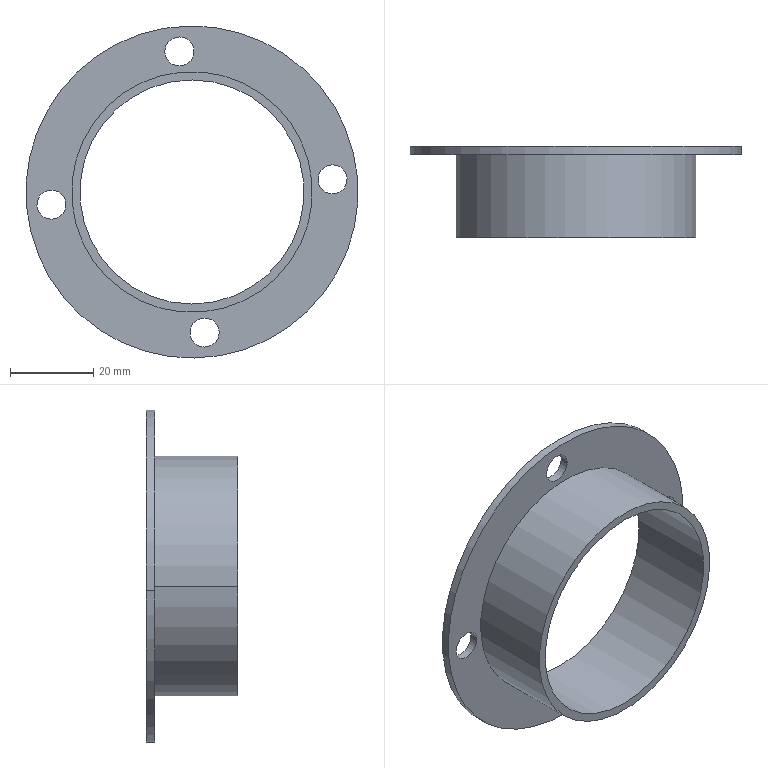Component | SolidWorks | ControllerRotatingShaft-1 | 1 solid | 17 faces | box 80 x 22 x 80 mm | volume 12202 mm3 | cylinder 14 | plane 3 | commonest cylinder face diameters 7 x8 80 x2 54 x2 58 x2
STEP:
#1=COLOUR_RGB('',0.7922,0.8196,0.9333);
#2=FILL_AREA_STYLE_COLOUR('',#1);
#3=FILL_AREA_STYLE('',(#2));
#4=SURFACE_STYLE_FILL_AREA(#3);
#5=SURFACE_SIDE_STYLE('',(#4));
#6=SURFACE_STYLE_USAGE(.BOTH.,#5);
#7=PRESENTATION_STYLE_ASSIGNMENT((#6));
#8=CARTESIAN_POINT('',(13.418,-5.647,18.276));
#9=VERTEX_POINT('',#8);
#10=CARTESIAN_POINT('',(13.693,-5.647,18.3));
#11=VERTEX_POINT('',#10);
#12=CARTESIAN_POINT('',(13.556,-5.647,18.288));
#13=DIRECTION('',(0.,1.,0.));
#14=DIRECTION('',(0.996,0.,0.08937));
#15=AXIS2_PLACEMENT_3D('',#12,#13,#14);
#16=CIRCLE('',#15,0.1378);
#17=EDGE_CURVE('',#9,#11,#16,.T.);
#18=ORIENTED_EDGE('',*,*,#17,.F.);
#19=CARTESIAN_POINT('',(13.418,-5.568,18.276));
#20=VERTEX_POINT('',#19);
#21=CARTESIAN_POINT('',(13.418,-5.962,18.276));
#22=DIRECTION('',(0.,1.,0.));
#23=VECTOR('',#22,39.37);
#24=LINE('',#21,#23);
#25=EDGE_CURVE('',#9,#20,#24,.T.);
#26=ORIENTED_EDGE('',*,*,#25,.T.);
#27=CARTESIAN_POINT('',(13.693,-5.568,18.3));
#28=VERTEX_POINT('',#27);
#29=CARTESIAN_POINT('',(13.556,-5.568,18.288));
#30=DIRECTION('',(0.,1.,0.));
#31=DIRECTION('',(-0.08937,0.,0.996));
#32=AXIS2_PLACEMENT_3D('',#29,#30,#31);
#33=CIRCLE('',#32,0.1378);
#34=EDGE_CURVE('',#20,#28,#33,.T.);
#35=ORIENTED_EDGE('',*,*,#34,.T.);
#36=CARTESIAN_POINT('',(13.693,-5.962,18.3));
#37=DIRECTION('',(0.,1.,0.));
#38=VECTOR('',#37,39.37);
#39=LINE('',#36,#38);
#40=EDGE_CURVE('',#11,#28,#39,.T.);
#41=ORIENTED_EDGE('',*,*,#40,.F.);
#42=EDGE_LOOP('',(#18,#26,#35,#41));
#43=FACE_OUTER_BOUND('',#42,.T.);
#44=CARTESIAN_POINT('',(13.556,-5.962,18.288));
#45=DIRECTION('',(0.,1.,0.));
#46=DIRECTION('',(0.996,0.,0.08937));
#47=AXIS2_PLACEMENT_3D('',#44,#45,#46);
#48=CYLINDRICAL_SURFACE('',#47,0.1378);
#49=ADVANCED_FACE('',(#43),#48,.F.);
#50=CARTESIAN_POINT('',(11.966,-5.647,19.489));
#51=VERTEX_POINT('',#50);
#52=CARTESIAN_POINT('',(12.24,-5.647,19.514));
#53=VERTEX_POINT('',#52);
#54=CARTESIAN_POINT('',(12.103,-5.647,19.502));
#55=DIRECTION('',(0.,1.,0.));
#56=DIRECTION('',(0.996,0.,0.08937));
#57=AXIS2_PLACEMENT_3D('',#54,#55,#56);
#58=CIRCLE('',#57,0.1378);
#59=EDGE_CURVE('',#51,#53,#58,.T.);
#60=ORIENTED_EDGE('',*,*,#59,.F.);
#61=CARTESIAN_POINT('',(11.966,-5.568,19.489));
#62=VERTEX_POINT('',#61);
#63=CARTESIAN_POINT('',(11.966,-5.962,19.489));
#64=DIRECTION('',(0.,1.,0.));
#65=VECTOR('',#64,39.37);
#66=LINE('',#63,#65);
#67=EDGE_CURVE('',#51,#62,#66,.T.);
#68=ORIENTED_EDGE('',*,*,#67,.T.);
#69=CARTESIAN_POINT('',(12.24,-5.568,19.514));
#70=VERTEX_POINT('',#69);
#71=CARTESIAN_POINT('',(12.103,-5.568,19.502));
#72=DIRECTION('',(0.,1.,0.));
#73=DIRECTION('',(-0.996,0.,-0.08937));
#74=AXIS2_PLACEMENT_3D('',#71,#72,#73);
#75=CIRCLE('',#74,0.1378);
#76=EDGE_CURVE('',#62,#70,#75,.T.);
#77=ORIENTED_EDGE('',*,*,#76,.T.);
#78=CARTESIAN_POINT('',(12.24,-5.962,19.514));
#79=DIRECTION('',(0.,1.,0.));
#80=VECTOR('',#79,39.37);
#81=LINE('',#78,#80);
#82=EDGE_CURVE('',#53,#70,#81,.T.);
#83=ORIENTED_EDGE('',*,*,#82,.F.);
#84=EDGE_LOOP('',(#60,#68,#77,#83));
#85=FACE_OUTER_BOUND('',#84,.T.);
#86=CARTESIAN_POINT('',(12.103,-5.962,19.502));
#87=DIRECTION('',(0.,1.,0.));
#88=DIRECTION('',(0.996,0.,0.08937));
#89=AXIS2_PLACEMENT_3D('',#86,#87,#88);
#90=CYLINDRICAL_SURFACE('',#89,0.1378);
#91=ADVANCED_FACE('',(#85),#90,.F.);
#92=CARTESIAN_POINT('',(10.752,-5.647,18.037));
#93=VERTEX_POINT('',#92);
#94=CARTESIAN_POINT('',(11.026,-5.647,18.061));
#95=VERTEX_POINT('',#94);
#96=CARTESIAN_POINT('',(10.889,-5.647,18.049));
#97=DIRECTION('',(0.,1.,0.));
#98=DIRECTION('',(0.996,0.,0.08937));
#99=AXIS2_PLACEMENT_3D('',#96,#97,#98);
#100=CIRCLE('',#99,0.1378);
#101=EDGE_CURVE('',#93,#95,#100,.T.);
#102=ORIENTED_EDGE('',*,*,#101,.F.);
#103=CARTESIAN_POINT('',(10.752,-5.568,18.037));
#104=VERTEX_POINT('',#103);
#105=CARTESIAN_POINT('',(10.752,-5.962,18.037));
#106=DIRECTION('',(0.,1.,0.));
#107=VECTOR('',#106,39.37);
#108=LINE('',#105,#107);
#109=EDGE_CURVE('',#93,#104,#108,.T.);
#110=ORIENTED_EDGE('',*,*,#109,.T.);
#111=CARTESIAN_POINT('',(11.026,-5.568,18.061));
#112=VERTEX_POINT('',#111);
#113=CARTESIAN_POINT('',(10.889,-5.568,18.049));
#114=DIRECTION('',(0.,1.,0.));
#115=DIRECTION('',(0.08937,0.,-0.996));
#116=AXIS2_PLACEMENT_3D('',#113,#114,#115);
#117=CIRCLE('',#116,0.1378);
#118=EDGE_CURVE('',#104,#112,#117,.T.);
#119=ORIENTED_EDGE('',*,*,#118,.T.);
#120=CARTESIAN_POINT('',(11.026,-5.962,18.061));
#121=DIRECTION('',(0.,1.,0.));
#122=VECTOR('',#121,39.37);
#123=LINE('',#120,#122);
#124=EDGE_CURVE('',#95,#112,#123,.T.);
#125=ORIENTED_EDGE('',*,*,#124,.F.);
#126=EDGE_LOOP('',(#102,#110,#119,#125));
#127=FACE_OUTER_BOUND('',#126,.T.);
#128=CARTESIAN_POINT('',(10.889,-5.962,18.049));
#129=DIRECTION('',(0.,1.,0.));
#130=DIRECTION('',(0.996,0.,0.08937));
#131=AXIS2_PLACEMENT_3D('',#128,#129,#130);
#132=CYLINDRICAL_SURFACE('',#131,0.1378);
#133=ADVANCED_FACE('',(#127),#132,.F.);
#134=CARTESIAN_POINT('',(12.205,-5.647,16.823));
#135=VERTEX_POINT('',#134);
#136=CARTESIAN_POINT('',(12.479,-5.647,16.848));
#137=VERTEX_POINT('',#136);
#138=CARTESIAN_POINT('',(12.342,-5.647,16.835));
#139=DIRECTION('',(0.,1.,0.));
#140=DIRECTION('',(0.996,0.,0.08937));
#141=AXIS2_PLACEMENT_3D('',#138,#139,#140);
#142=CIRCLE('',#141,0.1378);
#143=EDGE_CURVE('',#135,#137,#142,.T.);
#144=ORIENTED_EDGE('',*,*,#143,.F.);
#145=CARTESIAN_POINT('',(12.205,-5.568,16.823));
#146=VERTEX_POINT('',#145);
#147=CARTESIAN_POINT('',(12.205,-5.962,16.823));
#148=DIRECTION('',(0.,1.,0.));
#149=VECTOR('',#148,39.37);
#150=LINE('',#147,#149);
#151=EDGE_CURVE('',#135,#146,#150,.T.);
#152=ORIENTED_EDGE('',*,*,#151,.T.);
#153=CARTESIAN_POINT('',(12.479,-5.568,16.848));
#154=VERTEX_POINT('',#153);
#155=CARTESIAN_POINT('',(12.342,-5.568,16.835));
#156=DIRECTION('',(0.,1.,0.));
#157=DIRECTION('',(0.996,0.,0.08937));
#158=AXIS2_PLACEMENT_3D('',#155,#156,#157);
#159=CIRCLE('',#158,0.1378);
#160=EDGE_CURVE('',#146,#154,#159,.T.);
#161=ORIENTED_EDGE('',*,*,#160,.T.);
#162=CARTESIAN_POINT('',(12.479,-5.962,16.848));
#163=DIRECTION('',(0.,1.,0.));
#164=VECTOR('',#163,39.37);
#165=LINE('',#162,#164);
#166=EDGE_CURVE('',#137,#154,#165,.T.);
#167=ORIENTED_EDGE('',*,*,#166,.F.);
#168=EDGE_LOOP('',(#144,#152,#161,#167));
#169=FACE_OUTER_BOUND('',#168,.T.);
#170=CARTESIAN_POINT('',(12.342,-5.962,16.835));
#171=DIRECTION('',(0.,1.,0.));
#172=DIRECTION('',(0.996,0.,0.08937));
#173=AXIS2_PLACEMENT_3D('',#170,#171,#172);
#174=CYLINDRICAL_SURFACE('',#173,0.1378);
#175=ADVANCED_FACE('',(#169),#174,.F.);
#176=CARTESIAN_POINT('',(13.791,-5.568,18.309));
#177=VERTEX_POINT('',#176);
#178=CARTESIAN_POINT('',(10.654,-5.568,18.028));
#179=VERTEX_POINT('',#178);
#180=CARTESIAN_POINT('',(12.222,-5.568,18.169));
#181=DIRECTION('',(0.,1.,0.));
#182=DIRECTION('',(0.996,0.,0.08937));
#183=AXIS2_PLACEMENT_3D('',#180,#181,#182);
#184=CIRCLE('',#183,1.575);
#185=EDGE_CURVE('',#177,#179,#184,.T.);
#186=ORIENTED_EDGE('',*,*,#185,.F.);
#187=CARTESIAN_POINT('',(13.791,-5.647,18.309));
#188=VERTEX_POINT('',#187);
#189=CARTESIAN_POINT('',(13.791,-5.568,18.309));
#190=DIRECTION('',(-0.,-1.,-0.));
#191=VECTOR('',#190,39.37);
#192=LINE('',#189,#191);
#193=EDGE_CURVE('',#177,#188,#192,.T.);
#194=ORIENTED_EDGE('',*,*,#193,.T.);
#195=CARTESIAN_POINT('',(10.654,-5.647,18.028));
#196=VERTEX_POINT('',#195);
#197=CARTESIAN_POINT('',(12.222,-5.647,18.169));
#198=DIRECTION('',(0.,1.,0.));
#199=DIRECTION('',(0.996,0.,0.08937));
#200=AXIS2_PLACEMENT_3D('',#197,#198,#199);
#201=CIRCLE('',#200,1.575);
#202=EDGE_CURVE('',#188,#196,#201,.T.);
#203=ORIENTED_EDGE('',*,*,#202,.T.);
#204=CARTESIAN_POINT('',(10.654,-5.568,18.028));
#205=DIRECTION('',(-0.,-1.,-0.));
#206=VECTOR('',#205,39.37);
#207=LINE('',#204,#206);
#208=EDGE_CURVE('',#179,#196,#207,.T.);
#209=ORIENTED_EDGE('',*,*,#208,.F.);
#210=EDGE_LOOP('',(#186,#194,#203,#209));
#211=FACE_OUTER_BOUND('',#210,.T.);
#212=CARTESIAN_POINT('',(12.222,-5.568,18.169));
#213=DIRECTION('',(-0.,-1.,-0.));
#214=DIRECTION('',(-0.996,0.,-0.08937));
#215=AXIS2_PLACEMENT_3D('',#212,#213,#214);
#216=CYLINDRICAL_SURFACE('',#215,1.575);
#217=ADVANCED_FACE('',(#211),#216,.T.);
#218=CARTESIAN_POINT('',(11.164,-5.568,18.074));
#219=VERTEX_POINT('',#218);
#220=CARTESIAN_POINT('',(13.281,-5.568,18.264));
#221=VERTEX_POINT('',#220);
#222=CARTESIAN_POINT('',(12.222,-5.568,18.169));
#223=DIRECTION('',(0.,1.,0.));
#224=DIRECTION('',(0.996,0.,0.08937));
#225=AXIS2_PLACEMENT_3D('',#222,#223,#224);
#226=CIRCLE('',#225,1.063);
#227=EDGE_CURVE('',#219,#221,#226,.T.);
#228=ORIENTED_EDGE('',*,*,#227,.T.);
#229=CARTESIAN_POINT('',(13.281,-6.434,18.264));
#230=VERTEX_POINT('',#229);
#231=CARTESIAN_POINT('',(13.281,-5.647,18.264));
#232=DIRECTION('',(-0.,-1.,-0.));
#233=VECTOR('',#232,39.37);
#234=LINE('',#231,#233);
#235=EDGE_CURVE('',#221,#230,#234,.T.);
#236=ORIENTED_EDGE('',*,*,#235,.T.);
#237=CARTESIAN_POINT('',(11.164,-6.434,18.074));
#238=VERTEX_POINT('',#237);
#239=CARTESIAN_POINT('',(12.222,-6.434,18.169));
#240=DIRECTION('',(0.,1.,0.));
#241=DIRECTION('',(0.996,0.,0.08937));
#242=AXIS2_PLACEMENT_3D('',#239,#240,#241);
#243=CIRCLE('',#242,1.063);
#244=EDGE_CURVE('',#238,#230,#243,.T.);
#245=ORIENTED_EDGE('',*,*,#244,.F.);
#246=CARTESIAN_POINT('',(11.164,-5.647,18.074));
#247=DIRECTION('',(-0.,-1.,-0.));
#248=VECTOR('',#247,39.37);
#249=LINE('',#246,#248);
#250=EDGE_CURVE('',#219,#238,#249,.T.);
#251=ORIENTED_EDGE('',*,*,#250,.F.);
#252=EDGE_LOOP('',(#228,#236,#245,#251));
#253=FACE_OUTER_BOUND('',#252,.T.);
#254=CARTESIAN_POINT('',(12.222,-5.647,18.169));
#255=DIRECTION('',(-0.,-1.,-0.));
#256=DIRECTION('',(-0.996,0.,-0.08937));
#257=AXIS2_PLACEMENT_3D('',#254,#255,#256);
#258=CYLINDRICAL_SURFACE('',#257,1.063);
#259=ADVANCED_FACE('',(#253),#258,.F.);
#260=CARTESIAN_POINT('',(13.36,-5.647,18.271));
#261=VERTEX_POINT('',#260);
#262=CARTESIAN_POINT('',(11.085,-5.647,18.067));
#263=VERTEX_POINT('',#262);
#264=CARTESIAN_POINT('',(12.222,-5.647,18.169));
#265=DIRECTION('',(0.,1.,0.));
#266=DIRECTION('',(0.996,0.,0.08937));
#267=AXIS2_PLACEMENT_3D('',#264,#265,#266);
#268=CIRCLE('',#267,1.142);
#269=EDGE_CURVE('',#261,#263,#268,.T.);
#270=ORIENTED_EDGE('',*,*,#269,.F.);
#271=CARTESIAN_POINT('',(13.36,-6.434,18.271));
#272=VERTEX_POINT('',#271);
#273=CARTESIAN_POINT('',(13.36,-5.647,18.271));
#274=DIRECTION('',(-0.,-1.,-0.));
#275=VECTOR('',#274,39.37);
#276=LINE('',#273,#275);
#277=EDGE_CURVE('',#261,#272,#276,.T.);
#278=ORIENTED_EDGE('',*,*,#277,.T.);
#279=CARTESIAN_POINT('',(11.085,-6.434,18.067));
#280=VERTEX_POINT('',#279);
#281=CARTESIAN_POINT('',(12.222,-6.434,18.169));
#282=DIRECTION('',(0.,1.,0.));
#283=DIRECTION('',(0.996,0.,0.08937));
#284=AXIS2_PLACEMENT_3D('',#281,#282,#283);
#285=CIRCLE('',#284,1.142);
#286=EDGE_CURVE('',#272,#280,#285,.T.);
#287=ORIENTED_EDGE('',*,*,#286,.T.);
#288=CARTESIAN_POINT('',(11.085,-5.647,18.067));
#289=DIRECTION('',(-0.,-1.,-0.));
#290=VECTOR('',#289,39.37);
#291=LINE('',#288,#290);
#292=EDGE_CURVE('',#263,#280,#291,.T.);
#293=ORIENTED_EDGE('',*,*,#292,.F.);
#294=EDGE_LOOP('',(#270,#278,#287,#293));
#295=FACE_OUTER_BOUND('',#294,.T.);
#296=CARTESIAN_POINT('',(12.222,-5.647,18.169));
#297=DIRECTION('',(-0.,-1.,-0.));
#298=DIRECTION('',(-0.996,0.,-0.08937));
#299=AXIS2_PLACEMENT_3D('',#296,#297,#298);
#300=CYLINDRICAL_SURFACE('',#299,1.142);
#301=ADVANCED_FACE('',(#295),#300,.T.);
#302=CARTESIAN_POINT('',(12.222,-6.434,18.169));
#303=DIRECTION('',(0.,1.,0.));
#304=DIRECTION('',(0.996,0.,0.08937));
#305=AXIS2_PLACEMENT_3D('',#302,#303,#304);
#306=CIRCLE('',#305,1.142);
#307=EDGE_CURVE('',#280,#272,#306,.T.);
#308=ORIENTED_EDGE('',*,*,#307,.F.);
#309=ORIENTED_EDGE('',*,*,#286,.F.);
#310=EDGE_LOOP('',(#308,#309));
#311=FACE_OUTER_BOUND('',#310,.T.);
#312=ORIENTED_EDGE('',*,*,#244,.T.);
#313=CARTESIAN_POINT('',(12.222,-6.434,18.169));
#314=DIRECTION('',(0.,1.,0.));
#315=DIRECTION('',(0.996,0.,0.08937));
#316=AXIS2_PLACEMENT_3D('',#313,#314,#315);
#317=CIRCLE('',#316,1.063);
#318=EDGE_CURVE('',#230,#238,#317,.T.);
#319=ORIENTED_EDGE('',*,*,#318,.T.);
#320=EDGE_LOOP('',(#312,#319));
#321=FACE_BOUND('',#320,.T.);
#322=CARTESIAN_POINT('',(12.222,-6.434,18.169));
#323=DIRECTION('',(0.,1.,0.));
#324=DIRECTION('',(0.996,-0.,0.08937));
#325=AXIS2_PLACEMENT_3D('',#322,#323,#324);
#326=PLANE('',#325);
#327=ADVANCED_FACE('',(#311,#321),#326,.F.);
#328=ORIENTED_EDGE('',*,*,#277,.F.);
#329=CARTESIAN_POINT('',(12.222,-5.647,18.169));
#330=DIRECTION('',(0.,1.,0.));
#331=DIRECTION('',(0.996,0.,0.08937));
#332=AXIS2_PLACEMENT_3D('',#329,#330,#331);
#333=CIRCLE('',#332,1.142);
#334=EDGE_CURVE('',#263,#261,#333,.T.);
#335=ORIENTED_EDGE('',*,*,#334,.F.);
#336=ORIENTED_EDGE('',*,*,#292,.T.);
#337=ORIENTED_EDGE('',*,*,#307,.T.);
#338=EDGE_LOOP('',(#328,#335,#336,#337));
#339=FACE_OUTER_BOUND('',#338,.T.);
#340=CARTESIAN_POINT('',(12.222,-5.647,18.169));
#341=DIRECTION('',(-0.,-1.,-0.));
#342=DIRECTION('',(-0.996,0.,-0.08937));
#343=AXIS2_PLACEMENT_3D('',#340,#341,#342);
#344=CYLINDRICAL_SURFACE('',#343,1.142);
#345=ADVANCED_FACE('',(#339),#344,.T.);
#346=ORIENTED_EDGE('',*,*,#235,.F.);
#347=CARTESIAN_POINT('',(12.222,-5.568,18.169));
#348=DIRECTION('',(0.,1.,0.));
#349=DIRECTION('',(0.996,0.,0.08937));
#350=AXIS2_PLACEMENT_3D('',#347,#348,#349);
#351=CIRCLE('',#350,1.063);
#352=EDGE_CURVE('',#221,#219,#351,.T.);
#353=ORIENTED_EDGE('',*,*,#352,.T.);
#354=ORIENTED_EDGE('',*,*,#250,.T.);
#355=ORIENTED_EDGE('',*,*,#318,.F.);
#356=EDGE_LOOP('',(#346,#353,#354,#355));
#357=FACE_OUTER_BOUND('',#356,.T.);
#358=CARTESIAN_POINT('',(12.222,-5.647,18.169));
#359=DIRECTION('',(-0.,-1.,-0.));
#360=DIRECTION('',(-0.996,0.,-0.08937));
#361=AXIS2_PLACEMENT_3D('',#358,#359,#360);
#362=CYLINDRICAL_SURFACE('',#361,1.063);
#363=ADVANCED_FACE('',(#357),#362,.F.);
#364=CARTESIAN_POINT('',(13.556,-5.647,18.288));
#365=DIRECTION('',(0.,1.,0.));
#366=DIRECTION('',(0.996,0.,0.08937));
#367=AXIS2_PLACEMENT_3D('',#364,#365,#366);
#368=CIRCLE('',#367,0.1378);
#369=EDGE_CURVE('',#11,#9,#368,.T.);
#370=ORIENTED_EDGE('',*,*,#369,.T.);
#371=ORIENTED_EDGE('',*,*,#17,.T.);
#372=EDGE_LOOP('',(#370,#371));
#373=FACE_BOUND('',#372,.T.);
#374=CARTESIAN_POINT('',(12.103,-5.647,19.502));
#375=DIRECTION('',(0.,1.,0.));
#376=DIRECTION('',(0.996,0.,0.08937));
#377=AXIS2_PLACEMENT_3D('',#374,#375,#376);
#378=CIRCLE('',#377,0.1378);
#379=EDGE_CURVE('',#53,#51,#378,.T.);
#380=ORIENTED_EDGE('',*,*,#379,.T.);
#381=ORIENTED_EDGE('',*,*,#59,.T.);
#382=EDGE_LOOP('',(#380,#381));
#383=FACE_BOUND('',#382,.T.);
#384=CARTESIAN_POINT('',(10.889,-5.647,18.049));
#385=DIRECTION('',(0.,1.,0.));
#386=DIRECTION('',(0.996,0.,0.08937));
#387=AXIS2_PLACEMENT_3D('',#384,#385,#386);
#388=CIRCLE('',#387,0.1378);
#389=EDGE_CURVE('',#95,#93,#388,.T.);
#390=ORIENTED_EDGE('',*,*,#389,.T.);
#391=ORIENTED_EDGE('',*,*,#101,.T.);
#392=EDGE_LOOP('',(#390,#391));
#393=FACE_BOUND('',#392,.T.);
#394=CARTESIAN_POINT('',(12.342,-5.647,16.835));
#395=DIRECTION('',(0.,1.,0.));
#396=DIRECTION('',(0.996,0.,0.08937));
#397=AXIS2_PLACEMENT_3D('',#394,#395,#396);
#398=CIRCLE('',#397,0.1378);
#399=EDGE_CURVE('',#137,#135,#398,.T.);
#400=ORIENTED_EDGE('',*,*,#399,.T.);
#401=ORIENTED_EDGE('',*,*,#143,.T.);
#402=EDGE_LOOP('',(#400,#401));
#403=FACE_BOUND('',#402,.T.);
#404=CARTESIAN_POINT('',(12.222,-5.647,18.169));
#405=DIRECTION('',(0.,1.,0.));
#406=DIRECTION('',(0.996,0.,0.08937));
#407=AXIS2_PLACEMENT_3D('',#404,#405,#406);
#408=CIRCLE('',#407,1.575);
#409=EDGE_CURVE('',#196,#188,#408,.T.);
#410=ORIENTED_EDGE('',*,*,#409,.F.);
#411=ORIENTED_EDGE('',*,*,#202,.F.);
#412=EDGE_LOOP('',(#410,#411));
#413=FACE_OUTER_BOUND('',#412,.T.);
#414=ORIENTED_EDGE('',*,*,#334,.T.);
#415=ORIENTED_EDGE('',*,*,#269,.T.);
#416=EDGE_LOOP('',(#414,#415));
#417=FACE_BOUND('',#416,.T.);
#418=CARTESIAN_POINT('',(12.222,-5.647,18.169));
#419=DIRECTION('',(0.,1.,0.));
#420=DIRECTION('',(0.996,-0.,0.08937));
#421=AXIS2_PLACEMENT_3D('',#418,#419,#420);
#422=PLANE('',#421);
#423=ADVANCED_FACE('',(#373,#383,#393,#403,#413,#417),#422,.F.);
#424=CARTESIAN_POINT('',(13.556,-5.568,18.288));
#425=DIRECTION('',(0.,1.,0.));
#426=DIRECTION('',(-0.08937,0.,0.996));
#427=AXIS2_PLACEMENT_3D('',#424,#425,#426);
#428=CIRCLE('',#427,0.1378);
#429=EDGE_CURVE('',#28,#20,#428,.T.);
#430=ORIENTED_EDGE('',*,*,#429,.F.);
#431=ORIENTED_EDGE('',*,*,#34,.F.);
#432=EDGE_LOOP('',(#430,#431));
#433=FACE_BOUND('',#432,.T.);
#434=CARTESIAN_POINT('',(12.103,-5.568,19.502));
#435=DIRECTION('',(0.,1.,0.));
#436=DIRECTION('',(-0.996,0.,-0.08937));
#437=AXIS2_PLACEMENT_3D('',#434,#435,#436);
#438=CIRCLE('',#437,0.1378);
#439=EDGE_CURVE('',#70,#62,#438,.T.);
#440=ORIENTED_EDGE('',*,*,#439,.F.);
#441=ORIENTED_EDGE('',*,*,#76,.F.);
#442=EDGE_LOOP('',(#440,#441));
#443=FACE_BOUND('',#442,.T.);
#444=CARTESIAN_POINT('',(10.889,-5.568,18.049));
#445=DIRECTION('',(0.,1.,0.));
#446=DIRECTION('',(0.08937,0.,-0.996));
#447=AXIS2_PLACEMENT_3D('',#444,#445,#446);
#448=CIRCLE('',#447,0.1378);
#449=EDGE_CURVE('',#112,#104,#448,.T.);
#450=ORIENTED_EDGE('',*,*,#449,.F.);
#451=ORIENTED_EDGE('',*,*,#118,.F.);
#452=EDGE_LOOP('',(#450,#451));
#453=FACE_BOUND('',#452,.T.);
#454=CARTESIAN_POINT('',(12.342,-5.568,16.835));
#455=DIRECTION('',(0.,1.,0.));
#456=DIRECTION('',(0.996,0.,0.08937));
#457=AXIS2_PLACEMENT_3D('',#454,#455,#456);
#458=CIRCLE('',#457,0.1378);
#459=EDGE_CURVE('',#154,#146,#458,.T.);
#460=ORIENTED_EDGE('',*,*,#459,.F.);
#461=ORIENTED_EDGE('',*,*,#160,.F.);
#462=EDGE_LOOP('',(#460,#461));
#463=FACE_BOUND('',#462,.T.);
#464=CARTESIAN_POINT('',(12.222,-5.568,18.169));
#465=DIRECTION('',(0.,1.,0.));
#466=DIRECTION('',(0.996,0.,0.08937));
#467=AXIS2_PLACEMENT_3D('',#464,#465,#466);
#468=CIRCLE('',#467,1.575);
#469=EDGE_CURVE('',#179,#177,#468,.T.);
#470=ORIENTED_EDGE('',*,*,#469,.T.);
#471=ORIENTED_EDGE('',*,*,#185,.T.);
#472=EDGE_LOOP('',(#470,#471));
#473=FACE_OUTER_BOUND('',#472,.T.);
#474=ORIENTED_EDGE('',*,*,#227,.F.);
#475=ORIENTED_EDGE('',*,*,#352,.F.);
#476=EDGE_LOOP('',(#474,#475));
#477=FACE_BOUND('',#476,.T.);
#478=CARTESIAN_POINT('',(12.222,-5.568,18.169));
#479=DIRECTION('',(0.,1.,0.));
#480=DIRECTION('',(0.996,-0.,0.08937));
#481=AXIS2_PLACEMENT_3D('',#478,#479,#480);
#482=PLANE('',#481);
#483=ADVANCED_FACE('',(#433,#443,#453,#463,#473,#477),#482,.T.);
#484=ORIENTED_EDGE('',*,*,#193,.F.);
#485=ORIENTED_EDGE('',*,*,#469,.F.);
#486=ORIENTED_EDGE('',*,*,#208,.T.);
#487=ORIENTED_EDGE('',*,*,#409,.T.);
#488=EDGE_LOOP('',(#484,#485,#486,#487));
#489=FACE_OUTER_BOUND('',#488,.T.);
#490=CARTESIAN_POINT('',(12.222,-5.568,18.169));
#491=DIRECTION('',(-0.,-1.,-0.));
#492=DIRECTION('',(-0.996,0.,-0.08937));
#493=AXIS2_PLACEMENT_3D('',#490,#491,#492);
#494=CYLINDRICAL_SURFACE('',#493,1.575);
#495=ADVANCED_FACE('',(#489),#494,.T.);
#496=ORIENTED_EDGE('',*,*,#151,.F.);
#497=ORIENTED_EDGE('',*,*,#399,.F.);
#498=ORIENTED_EDGE('',*,*,#166,.T.);
#499=ORIENTED_EDGE('',*,*,#459,.T.);
#500=EDGE_LOOP('',(#496,#497,#498,#499));
#501=FACE_OUTER_BOUND('',#500,.T.);
#502=CARTESIAN_POINT('',(12.342,-5.962,16.835));
#503=DIRECTION('',(0.,1.,0.));
#504=DIRECTION('',(0.996,0.,0.08937));
#505=AXIS2_PLACEMENT_3D('',#502,#503,#504);
#506=CYLINDRICAL_SURFACE('',#505,0.1378);
#507=ADVANCED_FACE('',(#501),#506,.F.);
#508=ORIENTED_EDGE('',*,*,#109,.F.);
#509=ORIENTED_EDGE('',*,*,#389,.F.);
#510=ORIENTED_EDGE('',*,*,#124,.T.);
#511=ORIENTED_EDGE('',*,*,#449,.T.);
#512=EDGE_LOOP('',(#508,#509,#510,#511));
#513=FACE_OUTER_BOUND('',#512,.T.);
#514=CARTESIAN_POINT('',(10.889,-5.962,18.049));
#515=DIRECTION('',(0.,1.,0.));
#516=DIRECTION('',(0.996,0.,0.08937));
#517=AXIS2_PLACEMENT_3D('',#514,#515,#516);
#518=CYLINDRICAL_SURFACE('',#517,0.1378);
#519=ADVANCED_FACE('',(#513),#518,.F.);
#520=ORIENTED_EDGE('',*,*,#67,.F.);
#521=ORIENTED_EDGE('',*,*,#379,.F.);
#522=ORIENTED_EDGE('',*,*,#82,.T.);
#523=ORIENTED_EDGE('',*,*,#439,.T.);
#524=EDGE_LOOP('',(#520,#521,#522,#523));
#525=FACE_OUTER_BOUND('',#524,.T.);
#526=CARTESIAN_POINT('',(12.103,-5.962,19.502));
#527=DIRECTION('',(0.,1.,0.));
#528=DIRECTION('',(0.996,0.,0.08937));
#529=AXIS2_PLACEMENT_3D('',#526,#527,#528);
#530=CYLINDRICAL_SURFACE('',#529,0.1378);
#531=ADVANCED_FACE('',(#525),#530,.F.);
#532=ORIENTED_EDGE('',*,*,#25,.F.);
#533=ORIENTED_EDGE('',*,*,#369,.F.);
#534=ORIENTED_EDGE('',*,*,#40,.T.);
#535=ORIENTED_EDGE('',*,*,#429,.T.);
#536=EDGE_LOOP('',(#532,#533,#534,#535));
#537=FACE_OUTER_BOUND('',#536,.T.);
#538=CARTESIAN_POINT('',(13.556,-5.962,18.288));
#539=DIRECTION('',(0.,1.,0.));
#540=DIRECTION('',(0.996,0.,0.08937));
#541=AXIS2_PLACEMENT_3D('',#538,#539,#540);
#542=CYLINDRICAL_SURFACE('',#541,0.1378);
#543=ADVANCED_FACE('',(#537),#542,.F.);
#544=CLOSED_SHELL('',(#49,#91,#133,#175,#217,#259,#301,#327,#345,#363,#423,#483,#495,#507,#519,#531,#543));
#545=MANIFOLD_SOLID_BREP('',#544);
#546=STYLED_ITEM('',(#7),#545);
#547=PRESENTATION_LAYER_ASSIGNMENT('','',(#546));
#548=CARTESIAN_POINT('',(0.,0.,0.));
#549=DIRECTION('',(0.,0.,1.));
#550=DIRECTION('',(1.,0.,0.));
#551=AXIS2_PLACEMENT_3D('',#548,#549,#550);
#552=(LENGTH_UNIT()NAMED_UNIT(*)SI_UNIT($,.METRE.));
#553=LENGTH_MEASURE_WITH_UNIT(LENGTH_MEASURE(0.0254),#552);
#554=DIMENSIONAL_EXPONENTS(1.,0.,0.,0.,0.,0.,0.);
#555=(CONVERSION_BASED_UNIT('',#553)LENGTH_UNIT()NAMED_UNIT(#554));
#556=UNCERTAINTY_MEASURE_WITH_UNIT(LENGTH_MEASURE(0.00001),#555,'','');
#557=(NAMED_UNIT(*)PLANE_ANGLE_UNIT()SI_UNIT($,.RADIAN.));
#558=(NAMED_UNIT(*)SI_UNIT($,.STERADIAN.)SOLID_ANGLE_UNIT());
#559=(GEOMETRIC_REPRESENTATION_CONTEXT(3)GLOBAL_UNCERTAINTY_ASSIGNED_CONTEXT((#556))GLOBAL_UNIT_ASSIGNED_CONTEXT((#555,#557,#558))REPRESENTATION_CONTEXT('',''));
#560=ADVANCED_BREP_SHAPE_REPRESENTATION('',(#545,#551),#559);
#561=(LENGTH_UNIT()NAMED_UNIT(*)SI_UNIT($,.METRE.));
#562=LENGTH_MEASURE_WITH_UNIT(LENGTH_MEASURE(0.0254),#561);
#563=DIMENSIONAL_EXPONENTS(1.,0.,0.,0.,0.,0.,0.);
#564=(CONVERSION_BASED_UNIT('',#562)LENGTH_UNIT()NAMED_UNIT(#563));
#565=UNCERTAINTY_MEASURE_WITH_UNIT(LENGTH_MEASURE(0.00001),#564,'','');
#566=(NAMED_UNIT(*)PLANE_ANGLE_UNIT()SI_UNIT($,.RADIAN.));
#567=(NAMED_UNIT(*)SI_UNIT($,.STERADIAN.)SOLID_ANGLE_UNIT());
#568=(GEOMETRIC_REPRESENTATION_CONTEXT(3)GLOBAL_UNCERTAINTY_ASSIGNED_CONTEXT((#565))GLOBAL_UNIT_ASSIGNED_CONTEXT((#564,#566,#567))REPRESENTATION_CONTEXT('',''));
#569=MECHANICAL_DESIGN_GEOMETRIC_PRESENTATION_REPRESENTATION('',(#546),#568);